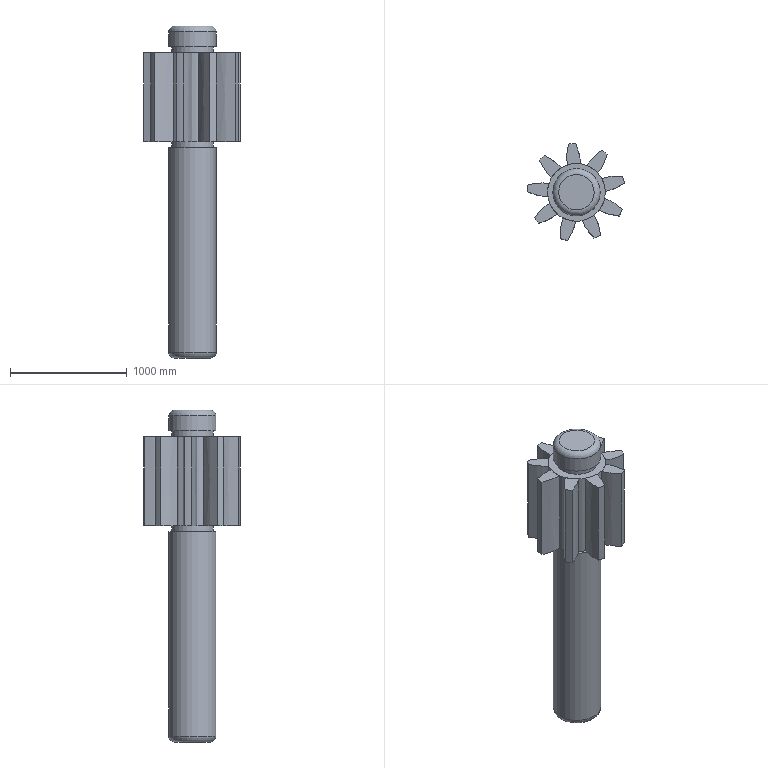Component | NX | 3 | 10 solids | 72 faces | volume 527427108 mm3 | plane 27 | cylinder 25 | other 18 | torus 2 | commonest cylinder face diameters 495.3 x10 838.2 x9 406.4 x2 355.6 x2 127 x2